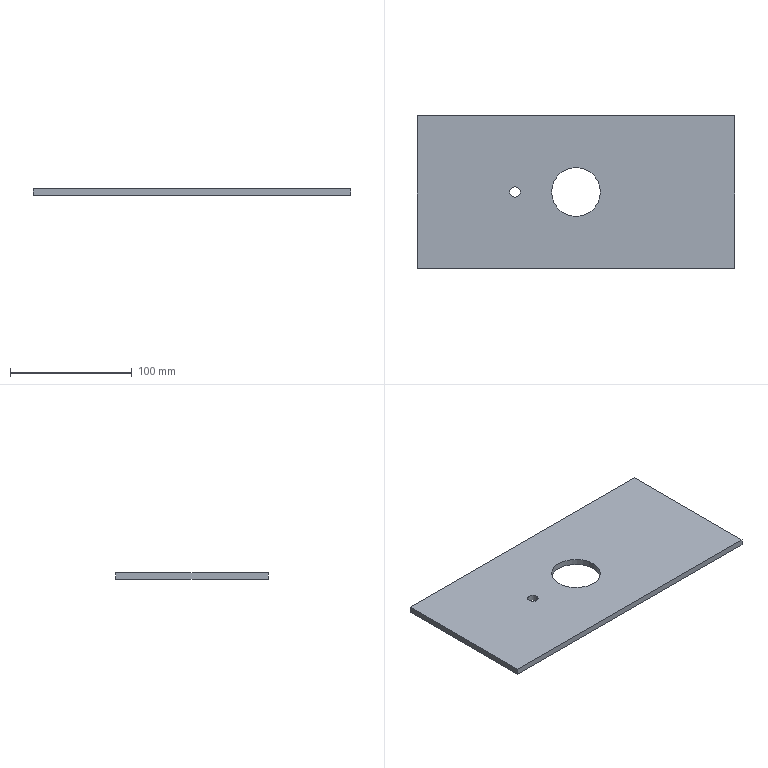Component | SolidWorks | 001LowerConnectingPlate-1 | 1 solid | 10 faces | box 260 x 125 x 5 mm | volume 155933 mm3 | plane 6 | cylinder 4 | commonest cylinder face diameters 8.5 x2 40 x2 | material Plain Carbon Steel
build123d program:
from build123d import *

# Parameters (mm, degrees)
SKETCH1_W              = 260
SKETCH1_H              = 125
BOSS_EXTRUDE1_DEPTH    = 5
CUT_EXTRUDE1_REACH     = 146.33
SKETCH2_R              = 20
M10_TAPPED_HOLE1_D     = 8.5
M10_TAPPED_HOLE1_DEPTH = 24.5
M10_TAPPED_HOLE1_TIP   = 2.554


with BuildPart() as part:
    # Sketch1 → Boss-Extrude1 (new body)
    with BuildSketch(Plane.XY):
        Rectangle(SKETCH1_W, SKETCH1_H)
    extrude(amount=BOSS_EXTRUDE1_DEPTH)

    # Sketch2 → Cut-Extrude1 (cut, up to next)
    with BuildSketch(Plane.XY.offset(5), mode=Mode.PRIVATE) as cut_extrude1_sk1:
        Circle(SKETCH2_R)
    cut_extrude1_tool1 = extrude(cut_extrude1_sk1.sketch, amount=-CUT_EXTRUDE1_REACH, mode=Mode.PRIVATE) & part.part
    add(cut_extrude1_tool1.solids().sort_by_distance((0, 0, 5))[0], mode=Mode.SUBTRACT)

    # M10 Tapped Hole1
    with Locations(Plane.XY.offset(5)):
        with Locations((50, 0)):
            Hole(M10_TAPPED_HOLE1_D / 2, depth=M10_TAPPED_HOLE1_DEPTH)
            with Locations((0, 0, -(M10_TAPPED_HOLE1_DEPTH + M10_TAPPED_HOLE1_TIP / 2))):  # 118° drill point
                Cone(0, M10_TAPPED_HOLE1_D / 2, M10_TAPPED_HOLE1_TIP, mode=Mode.SUBTRACT)


solid = part.part

# Placed as in the assembly
solid = solid.moved(Location((130, 99.5, -515), (-180, 0, 180)))
STEP:
#1=CARTESIAN_POINT('',(2.982,3.917,-20.276));
#2=VERTEX_POINT('',#1);
#3=CARTESIAN_POINT('',(3.317,3.917,-20.276));
#4=VERTEX_POINT('',#3);
#5=CARTESIAN_POINT('',(3.15,3.917,-20.276));
#6=DIRECTION('',(0.,0.,1.));
#7=DIRECTION('',(1.,0.,0.));
#8=AXIS2_PLACEMENT_3D('',#5,#6,#7);
#9=CIRCLE('',#8,0.1673);
#10=EDGE_CURVE('',#2,#4,#9,.T.);
#11=ORIENTED_EDGE('',*,*,#10,.T.);
#12=CARTESIAN_POINT('',(3.317,3.917,-20.472));
#13=VERTEX_POINT('',#12);
#14=CARTESIAN_POINT('',(3.317,3.917,-20.472));
#15=DIRECTION('',(0.,0.,-1.));
#16=VECTOR('',#15,39.37);
#17=LINE('',#14,#16);
#18=EDGE_CURVE('',#4,#13,#17,.T.);
#19=ORIENTED_EDGE('',*,*,#18,.T.);
#20=CARTESIAN_POINT('',(2.982,3.917,-20.472));
#21=VERTEX_POINT('',#20);
#22=CARTESIAN_POINT('',(3.15,3.917,-20.472));
#23=DIRECTION('',(0.,0.,-1.));
#24=DIRECTION('',(-1.,0.,0.));
#25=AXIS2_PLACEMENT_3D('',#22,#23,#24);
#26=CIRCLE('',#25,0.1673);
#27=EDGE_CURVE('',#13,#21,#26,.T.);
#28=ORIENTED_EDGE('',*,*,#27,.T.);
#29=CARTESIAN_POINT('',(2.982,3.917,-20.472));
#30=DIRECTION('',(0.,0.,-1.));
#31=VECTOR('',#30,39.37);
#32=LINE('',#29,#31);
#33=EDGE_CURVE('',#2,#21,#32,.T.);
#34=ORIENTED_EDGE('',*,*,#33,.F.);
#35=EDGE_LOOP('',(#11,#19,#28,#34));
#36=FACE_OUTER_BOUND('',#35,.T.);
#37=CARTESIAN_POINT('',(3.15,3.917,-20.472));
#38=DIRECTION('',(0.,0.,-1.));
#39=DIRECTION('',(-1.,0.,0.));
#40=AXIS2_PLACEMENT_3D('',#37,#38,#39);
#41=CYLINDRICAL_SURFACE('',#40,0.1673);
#42=ADVANCED_FACE('',(#36),#41,.F.);
#43=CARTESIAN_POINT('',(5.906,3.917,-20.276));
#44=VERTEX_POINT('',#43);
#45=CARTESIAN_POINT('',(4.331,3.917,-20.276));
#46=VERTEX_POINT('',#45);
#47=CARTESIAN_POINT('',(5.118,3.917,-20.276));
#48=DIRECTION('',(0.,0.,-1.));
#49=DIRECTION('',(1.,0.,0.));
#50=AXIS2_PLACEMENT_3D('',#47,#48,#49);
#51=CIRCLE('',#50,0.7874);
#52=EDGE_CURVE('',#44,#46,#51,.T.);
#53=ORIENTED_EDGE('',*,*,#52,.F.);
#54=CARTESIAN_POINT('',(5.906,3.917,-20.472));
#55=VERTEX_POINT('',#54);
#56=CARTESIAN_POINT('',(5.906,3.917,-20.276));
#57=DIRECTION('',(0.,0.,-1.));
#58=VECTOR('',#57,39.37);
#59=LINE('',#56,#58);
#60=EDGE_CURVE('',#44,#55,#59,.T.);
#61=ORIENTED_EDGE('',*,*,#60,.T.);
#62=CARTESIAN_POINT('',(4.331,3.917,-20.472));
#63=VERTEX_POINT('',#62);
#64=CARTESIAN_POINT('',(5.118,3.917,-20.472));
#65=DIRECTION('',(0.,0.,-1.));
#66=DIRECTION('',(-1.,0.,0.));
#67=AXIS2_PLACEMENT_3D('',#64,#65,#66);
#68=CIRCLE('',#67,0.7874);
#69=EDGE_CURVE('',#55,#63,#68,.T.);
#70=ORIENTED_EDGE('',*,*,#69,.T.);
#71=CARTESIAN_POINT('',(4.331,3.917,-20.276));
#72=DIRECTION('',(0.,0.,-1.));
#73=VECTOR('',#72,39.37);
#74=LINE('',#71,#73);
#75=EDGE_CURVE('',#46,#63,#74,.T.);
#76=ORIENTED_EDGE('',*,*,#75,.F.);
#77=EDGE_LOOP('',(#53,#61,#70,#76));
#78=FACE_OUTER_BOUND('',#77,.T.);
#79=CARTESIAN_POINT('',(5.118,3.917,-20.276));
#80=DIRECTION('',(0.,0.,-1.));
#81=DIRECTION('',(-1.,0.,0.));
#82=AXIS2_PLACEMENT_3D('',#79,#80,#81);
#83=CYLINDRICAL_SURFACE('',#82,0.7874);
#84=ADVANCED_FACE('',(#78),#83,.F.);
#85=CARTESIAN_POINT('',(0.,1.457,-20.276));
#86=VERTEX_POINT('',#85);
#87=CARTESIAN_POINT('',(0.,6.378,-20.276));
#88=VERTEX_POINT('',#87);
#89=CARTESIAN_POINT('',(0.,1.457,-20.276));
#90=DIRECTION('',(-0.,1.,0.));
#91=VECTOR('',#90,39.37);
#92=LINE('',#89,#91);
#93=EDGE_CURVE('',#86,#88,#92,.T.);
#94=ORIENTED_EDGE('',*,*,#93,.T.);
#95=CARTESIAN_POINT('',(0.,6.378,-20.472));
#96=VERTEX_POINT('',#95);
#97=CARTESIAN_POINT('',(0.,6.378,-20.472));
#98=DIRECTION('',(0.,0.,1.));
#99=VECTOR('',#98,39.37);
#100=LINE('',#97,#99);
#101=EDGE_CURVE('',#96,#88,#100,.T.);
#102=ORIENTED_EDGE('',*,*,#101,.F.);
#103=CARTESIAN_POINT('',(0.,1.457,-20.472));
#104=VERTEX_POINT('',#103);
#105=CARTESIAN_POINT('',(0.,1.457,-20.472));
#106=DIRECTION('',(-0.,1.,0.));
#107=VECTOR('',#106,39.37);
#108=LINE('',#105,#107);
#109=EDGE_CURVE('',#104,#96,#108,.T.);
#110=ORIENTED_EDGE('',*,*,#109,.F.);
#111=CARTESIAN_POINT('',(0.,1.457,-20.472));
#112=DIRECTION('',(0.,0.,1.));
#113=VECTOR('',#112,39.37);
#114=LINE('',#111,#113);
#115=EDGE_CURVE('',#104,#86,#114,.T.);
#116=ORIENTED_EDGE('',*,*,#115,.T.);
#117=EDGE_LOOP('',(#94,#102,#110,#116));
#118=FACE_OUTER_BOUND('',#117,.T.);
#119=CARTESIAN_POINT('',(0.,1.457,-20.472));
#120=DIRECTION('',(1.,0.,0.));
#121=DIRECTION('',(0.,0.,-1.));
#122=AXIS2_PLACEMENT_3D('',#119,#120,#121);
#123=PLANE('',#122);
#124=ADVANCED_FACE('',(#118),#123,.F.);
#125=CARTESIAN_POINT('',(10.236,6.378,-20.276));
#126=VERTEX_POINT('',#125);
#127=CARTESIAN_POINT('',(10.236,6.378,-20.276));
#128=DIRECTION('',(1.,0.,0.));
#129=VECTOR('',#128,39.37);
#130=LINE('',#127,#129);
#131=EDGE_CURVE('',#88,#126,#130,.T.);
#132=ORIENTED_EDGE('',*,*,#131,.T.);
#133=CARTESIAN_POINT('',(10.236,6.378,-20.472));
#134=VERTEX_POINT('',#133);
#135=CARTESIAN_POINT('',(10.236,6.378,-20.472));
#136=DIRECTION('',(0.,0.,1.));
#137=VECTOR('',#136,39.37);
#138=LINE('',#135,#137);
#139=EDGE_CURVE('',#134,#126,#138,.T.);
#140=ORIENTED_EDGE('',*,*,#139,.F.);
#141=CARTESIAN_POINT('',(10.236,6.378,-20.472));
#142=DIRECTION('',(1.,0.,0.));
#143=VECTOR('',#142,39.37);
#144=LINE('',#141,#143);
#145=EDGE_CURVE('',#96,#134,#144,.T.);
#146=ORIENTED_EDGE('',*,*,#145,.F.);
#147=ORIENTED_EDGE('',*,*,#101,.T.);
#148=EDGE_LOOP('',(#132,#140,#146,#147));
#149=FACE_OUTER_BOUND('',#148,.T.);
#150=CARTESIAN_POINT('',(10.236,6.378,-20.472));
#151=DIRECTION('',(0.,-1.,0.));
#152=DIRECTION('',(0.,0.,1.));
#153=AXIS2_PLACEMENT_3D('',#150,#151,#152);
#154=PLANE('',#153);
#155=ADVANCED_FACE('',(#149),#154,.F.);
#156=CARTESIAN_POINT('',(10.236,1.457,-20.276));
#157=VERTEX_POINT('',#156);
#158=CARTESIAN_POINT('',(10.236,1.457,-20.276));
#159=DIRECTION('',(0.,-1.,0.));
#160=VECTOR('',#159,39.37);
#161=LINE('',#158,#160);
#162=EDGE_CURVE('',#126,#157,#161,.T.);
#163=ORIENTED_EDGE('',*,*,#162,.T.);
#164=CARTESIAN_POINT('',(10.236,1.457,-20.472));
#165=VERTEX_POINT('',#164);
#166=CARTESIAN_POINT('',(10.236,1.457,-20.472));
#167=DIRECTION('',(0.,0.,1.));
#168=VECTOR('',#167,39.37);
#169=LINE('',#166,#168);
#170=EDGE_CURVE('',#165,#157,#169,.T.);
#171=ORIENTED_EDGE('',*,*,#170,.F.);
#172=CARTESIAN_POINT('',(10.236,1.457,-20.472));
#173=DIRECTION('',(0.,-1.,0.));
#174=VECTOR('',#173,39.37);
#175=LINE('',#172,#174);
#176=EDGE_CURVE('',#134,#165,#175,.T.);
#177=ORIENTED_EDGE('',*,*,#176,.F.);
#178=ORIENTED_EDGE('',*,*,#139,.T.);
#179=EDGE_LOOP('',(#163,#171,#177,#178));
#180=FACE_OUTER_BOUND('',#179,.T.);
#181=CARTESIAN_POINT('',(10.236,1.457,-20.472));
#182=DIRECTION('',(-1.,0.,0.));
#183=DIRECTION('',(0.,0.,1.));
#184=AXIS2_PLACEMENT_3D('',#181,#182,#183);
#185=PLANE('',#184);
#186=ADVANCED_FACE('',(#180),#185,.F.);
#187=CARTESIAN_POINT('',(10.236,1.457,-20.276));
#188=DIRECTION('',(-1.,0.,0.));
#189=VECTOR('',#188,39.37);
#190=LINE('',#187,#189);
#191=EDGE_CURVE('',#157,#86,#190,.T.);
#192=ORIENTED_EDGE('',*,*,#191,.T.);
#193=ORIENTED_EDGE('',*,*,#115,.F.);
#194=CARTESIAN_POINT('',(10.236,1.457,-20.472));
#195=DIRECTION('',(-1.,0.,0.));
#196=VECTOR('',#195,39.37);
#197=LINE('',#194,#196);
#198=EDGE_CURVE('',#165,#104,#197,.T.);
#199=ORIENTED_EDGE('',*,*,#198,.F.);
#200=ORIENTED_EDGE('',*,*,#170,.T.);
#201=EDGE_LOOP('',(#192,#193,#199,#200));
#202=FACE_OUTER_BOUND('',#201,.T.);
#203=CARTESIAN_POINT('',(10.236,1.457,-20.472));
#204=DIRECTION('',(-0.,1.,0.));
#205=DIRECTION('',(0.,0.,-1.));
#206=AXIS2_PLACEMENT_3D('',#203,#204,#205);
#207=PLANE('',#206);
#208=ADVANCED_FACE('',(#202),#207,.F.);
#209=CARTESIAN_POINT('',(3.15,3.917,-20.472));
#210=DIRECTION('',(0.,0.,-1.));
#211=DIRECTION('',(-1.,0.,0.));
#212=AXIS2_PLACEMENT_3D('',#209,#210,#211);
#213=CIRCLE('',#212,0.1673);
#214=EDGE_CURVE('',#21,#13,#213,.T.);
#215=ORIENTED_EDGE('',*,*,#214,.F.);
#216=ORIENTED_EDGE('',*,*,#27,.F.);
#217=EDGE_LOOP('',(#215,#216));
#218=FACE_BOUND('',#217,.T.);
#219=CARTESIAN_POINT('',(5.118,3.917,-20.472));
#220=DIRECTION('',(0.,0.,-1.));
#221=DIRECTION('',(-1.,0.,0.));
#222=AXIS2_PLACEMENT_3D('',#219,#220,#221);
#223=CIRCLE('',#222,0.7874);
#224=EDGE_CURVE('',#63,#55,#223,.T.);
#225=ORIENTED_EDGE('',*,*,#224,.F.);
#226=ORIENTED_EDGE('',*,*,#69,.F.);
#227=EDGE_LOOP('',(#225,#226));
#228=FACE_BOUND('',#227,.T.);
#229=ORIENTED_EDGE('',*,*,#109,.T.);
#230=ORIENTED_EDGE('',*,*,#145,.T.);
#231=ORIENTED_EDGE('',*,*,#176,.T.);
#232=ORIENTED_EDGE('',*,*,#198,.T.);
#233=EDGE_LOOP('',(#229,#230,#231,#232));
#234=FACE_OUTER_BOUND('',#233,.T.);
#235=CARTESIAN_POINT('',(0.,6.378,-20.472));
#236=DIRECTION('',(0.,0.,1.));
#237=DIRECTION('',(1.,0.,0.));
#238=AXIS2_PLACEMENT_3D('',#235,#236,#237);
#239=PLANE('',#238);
#240=ADVANCED_FACE('',(#218,#228,#234),#239,.F.);
#241=ORIENTED_EDGE('',*,*,#10,.F.);
#242=CARTESIAN_POINT('',(3.15,3.917,-20.276));
#243=DIRECTION('',(0.,0.,1.));
#244=DIRECTION('',(1.,0.,0.));
#245=AXIS2_PLACEMENT_3D('',#242,#243,#244);
#246=CIRCLE('',#245,0.1673);
#247=EDGE_CURVE('',#4,#2,#246,.T.);
#248=ORIENTED_EDGE('',*,*,#247,.F.);
#249=EDGE_LOOP('',(#241,#248));
#250=FACE_BOUND('',#249,.T.);
#251=CARTESIAN_POINT('',(5.118,3.917,-20.276));
#252=DIRECTION('',(0.,0.,-1.));
#253=DIRECTION('',(1.,0.,0.));
#254=AXIS2_PLACEMENT_3D('',#251,#252,#253);
#255=CIRCLE('',#254,0.7874);
#256=EDGE_CURVE('',#46,#44,#255,.T.);
#257=ORIENTED_EDGE('',*,*,#256,.T.);
#258=ORIENTED_EDGE('',*,*,#52,.T.);
#259=EDGE_LOOP('',(#257,#258));
#260=FACE_BOUND('',#259,.T.);
#261=ORIENTED_EDGE('',*,*,#93,.F.);
#262=ORIENTED_EDGE('',*,*,#191,.F.);
#263=ORIENTED_EDGE('',*,*,#162,.F.);
#264=ORIENTED_EDGE('',*,*,#131,.F.);
#265=EDGE_LOOP('',(#261,#262,#263,#264));
#266=FACE_OUTER_BOUND('',#265,.T.);
#267=CARTESIAN_POINT('',(0.,6.378,-20.276));
#268=DIRECTION('',(0.,0.,1.));
#269=DIRECTION('',(1.,0.,0.));
#270=AXIS2_PLACEMENT_3D('',#267,#268,#269);
#271=PLANE('',#270);
#272=ADVANCED_FACE('',(#250,#260,#266),#271,.T.);
#273=ORIENTED_EDGE('',*,*,#60,.F.);
#274=ORIENTED_EDGE('',*,*,#256,.F.);
#275=ORIENTED_EDGE('',*,*,#75,.T.);
#276=ORIENTED_EDGE('',*,*,#224,.T.);
#277=EDGE_LOOP('',(#273,#274,#275,#276));
#278=FACE_OUTER_BOUND('',#277,.T.);
#279=CARTESIAN_POINT('',(5.118,3.917,-20.276));
#280=DIRECTION('',(0.,0.,-1.));
#281=DIRECTION('',(-1.,0.,0.));
#282=AXIS2_PLACEMENT_3D('',#279,#280,#281);
#283=CYLINDRICAL_SURFACE('',#282,0.7874);
#284=ADVANCED_FACE('',(#278),#283,.F.);
#285=ORIENTED_EDGE('',*,*,#18,.F.);
#286=ORIENTED_EDGE('',*,*,#247,.T.);
#287=ORIENTED_EDGE('',*,*,#33,.T.);
#288=ORIENTED_EDGE('',*,*,#214,.T.);
#289=EDGE_LOOP('',(#285,#286,#287,#288));
#290=FACE_OUTER_BOUND('',#289,.T.);
#291=CARTESIAN_POINT('',(3.15,3.917,-20.472));
#292=DIRECTION('',(0.,0.,-1.));
#293=DIRECTION('',(-1.,0.,0.));
#294=AXIS2_PLACEMENT_3D('',#291,#292,#293);
#295=CYLINDRICAL_SURFACE('',#294,0.1673);
#296=ADVANCED_FACE('',(#290),#295,.F.);
#297=CLOSED_SHELL('',(#42,#84,#124,#155,#186,#208,#240,#272,#284,#296));
#298=MANIFOLD_SOLID_BREP('',#297);
#299=CARTESIAN_POINT('',(0.,0.,0.));
#300=DIRECTION('',(0.,0.,1.));
#301=DIRECTION('',(1.,0.,0.));
#302=AXIS2_PLACEMENT_3D('',#299,#300,#301);
#303=(LENGTH_UNIT()NAMED_UNIT(*)SI_UNIT($,.METRE.));
#304=LENGTH_MEASURE_WITH_UNIT(LENGTH_MEASURE(0.0254),#303);
#305=DIMENSIONAL_EXPONENTS(1.,0.,0.,0.,0.,0.,0.);
#306=(CONVERSION_BASED_UNIT('',#304)LENGTH_UNIT()NAMED_UNIT(#305));
#307=UNCERTAINTY_MEASURE_WITH_UNIT(LENGTH_MEASURE(0.00001),#306,'','');
#308=(NAMED_UNIT(*)PLANE_ANGLE_UNIT()SI_UNIT($,.RADIAN.));
#309=(NAMED_UNIT(*)SI_UNIT($,.STERADIAN.)SOLID_ANGLE_UNIT());
#310=(GEOMETRIC_REPRESENTATION_CONTEXT(3)GLOBAL_UNCERTAINTY_ASSIGNED_CONTEXT((#307))GLOBAL_UNIT_ASSIGNED_CONTEXT((#306,#308,#309))REPRESENTATION_CONTEXT('',''));
#311=ADVANCED_BREP_SHAPE_REPRESENTATION('',(#298,#302),#310);
#312=COLOUR_RGB('',0.7922,0.8196,0.9333);
#313=FILL_AREA_STYLE_COLOUR('',#312);
#314=FILL_AREA_STYLE('',(#313));
#315=SURFACE_STYLE_FILL_AREA(#314);
#316=SURFACE_SIDE_STYLE('',(#315));
#317=SURFACE_STYLE_USAGE(.BOTH.,#316);
#318=PRESENTATION_STYLE_ASSIGNMENT((#317));
#319=STYLED_ITEM('',(#318),#298);
#320=PRESENTATION_LAYER_ASSIGNMENT('','',(#319));
#321=(LENGTH_UNIT()NAMED_UNIT(*)SI_UNIT($,.METRE.));
#322=LENGTH_MEASURE_WITH_UNIT(LENGTH_MEASURE(0.0254),#321);
#323=DIMENSIONAL_EXPONENTS(1.,0.,0.,0.,0.,0.,0.);
#324=(CONVERSION_BASED_UNIT('',#322)LENGTH_UNIT()NAMED_UNIT(#323));
#325=UNCERTAINTY_MEASURE_WITH_UNIT(LENGTH_MEASURE(0.00001),#324,'','');
#326=(NAMED_UNIT(*)PLANE_ANGLE_UNIT()SI_UNIT($,.RADIAN.));
#327=(NAMED_UNIT(*)SI_UNIT($,.STERADIAN.)SOLID_ANGLE_UNIT());
#328=(GEOMETRIC_REPRESENTATION_CONTEXT(3)GLOBAL_UNCERTAINTY_ASSIGNED_CONTEXT((#325))GLOBAL_UNIT_ASSIGNED_CONTEXT((#324,#326,#327))REPRESENTATION_CONTEXT('',''));
#329=MECHANICAL_DESIGN_GEOMETRIC_PRESENTATION_REPRESENTATION('',(#319),#328);